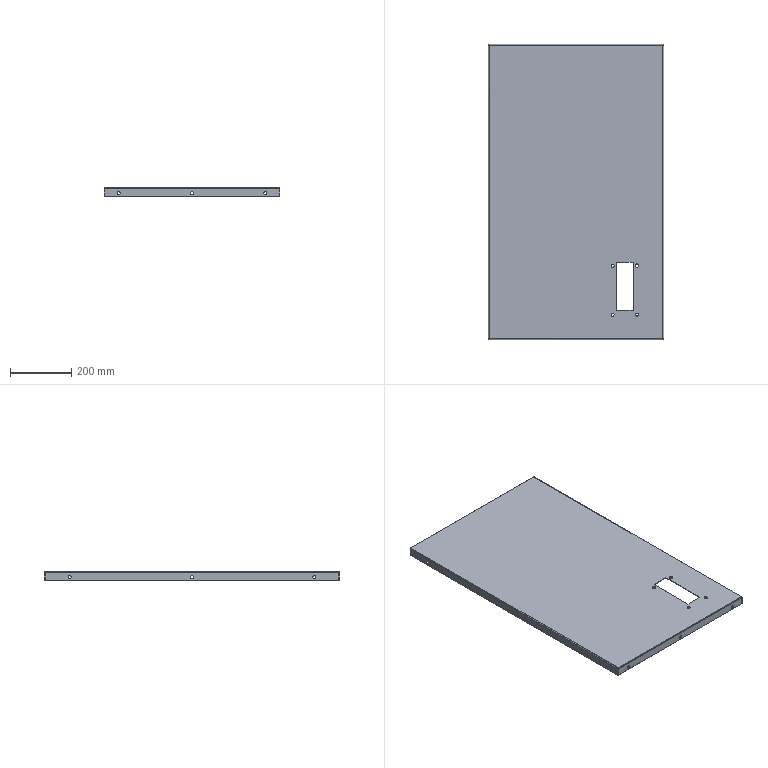Component | SolidWorks | 33FrontDoorUpperRightPlate-1 | 1 solid | 74 faces | volume 1243872 mm3 | cylinder 40 | plane 26 | spline 8 | commonest cylinder face diameters 10 x30 2 x4 6 x4 11.308 x2